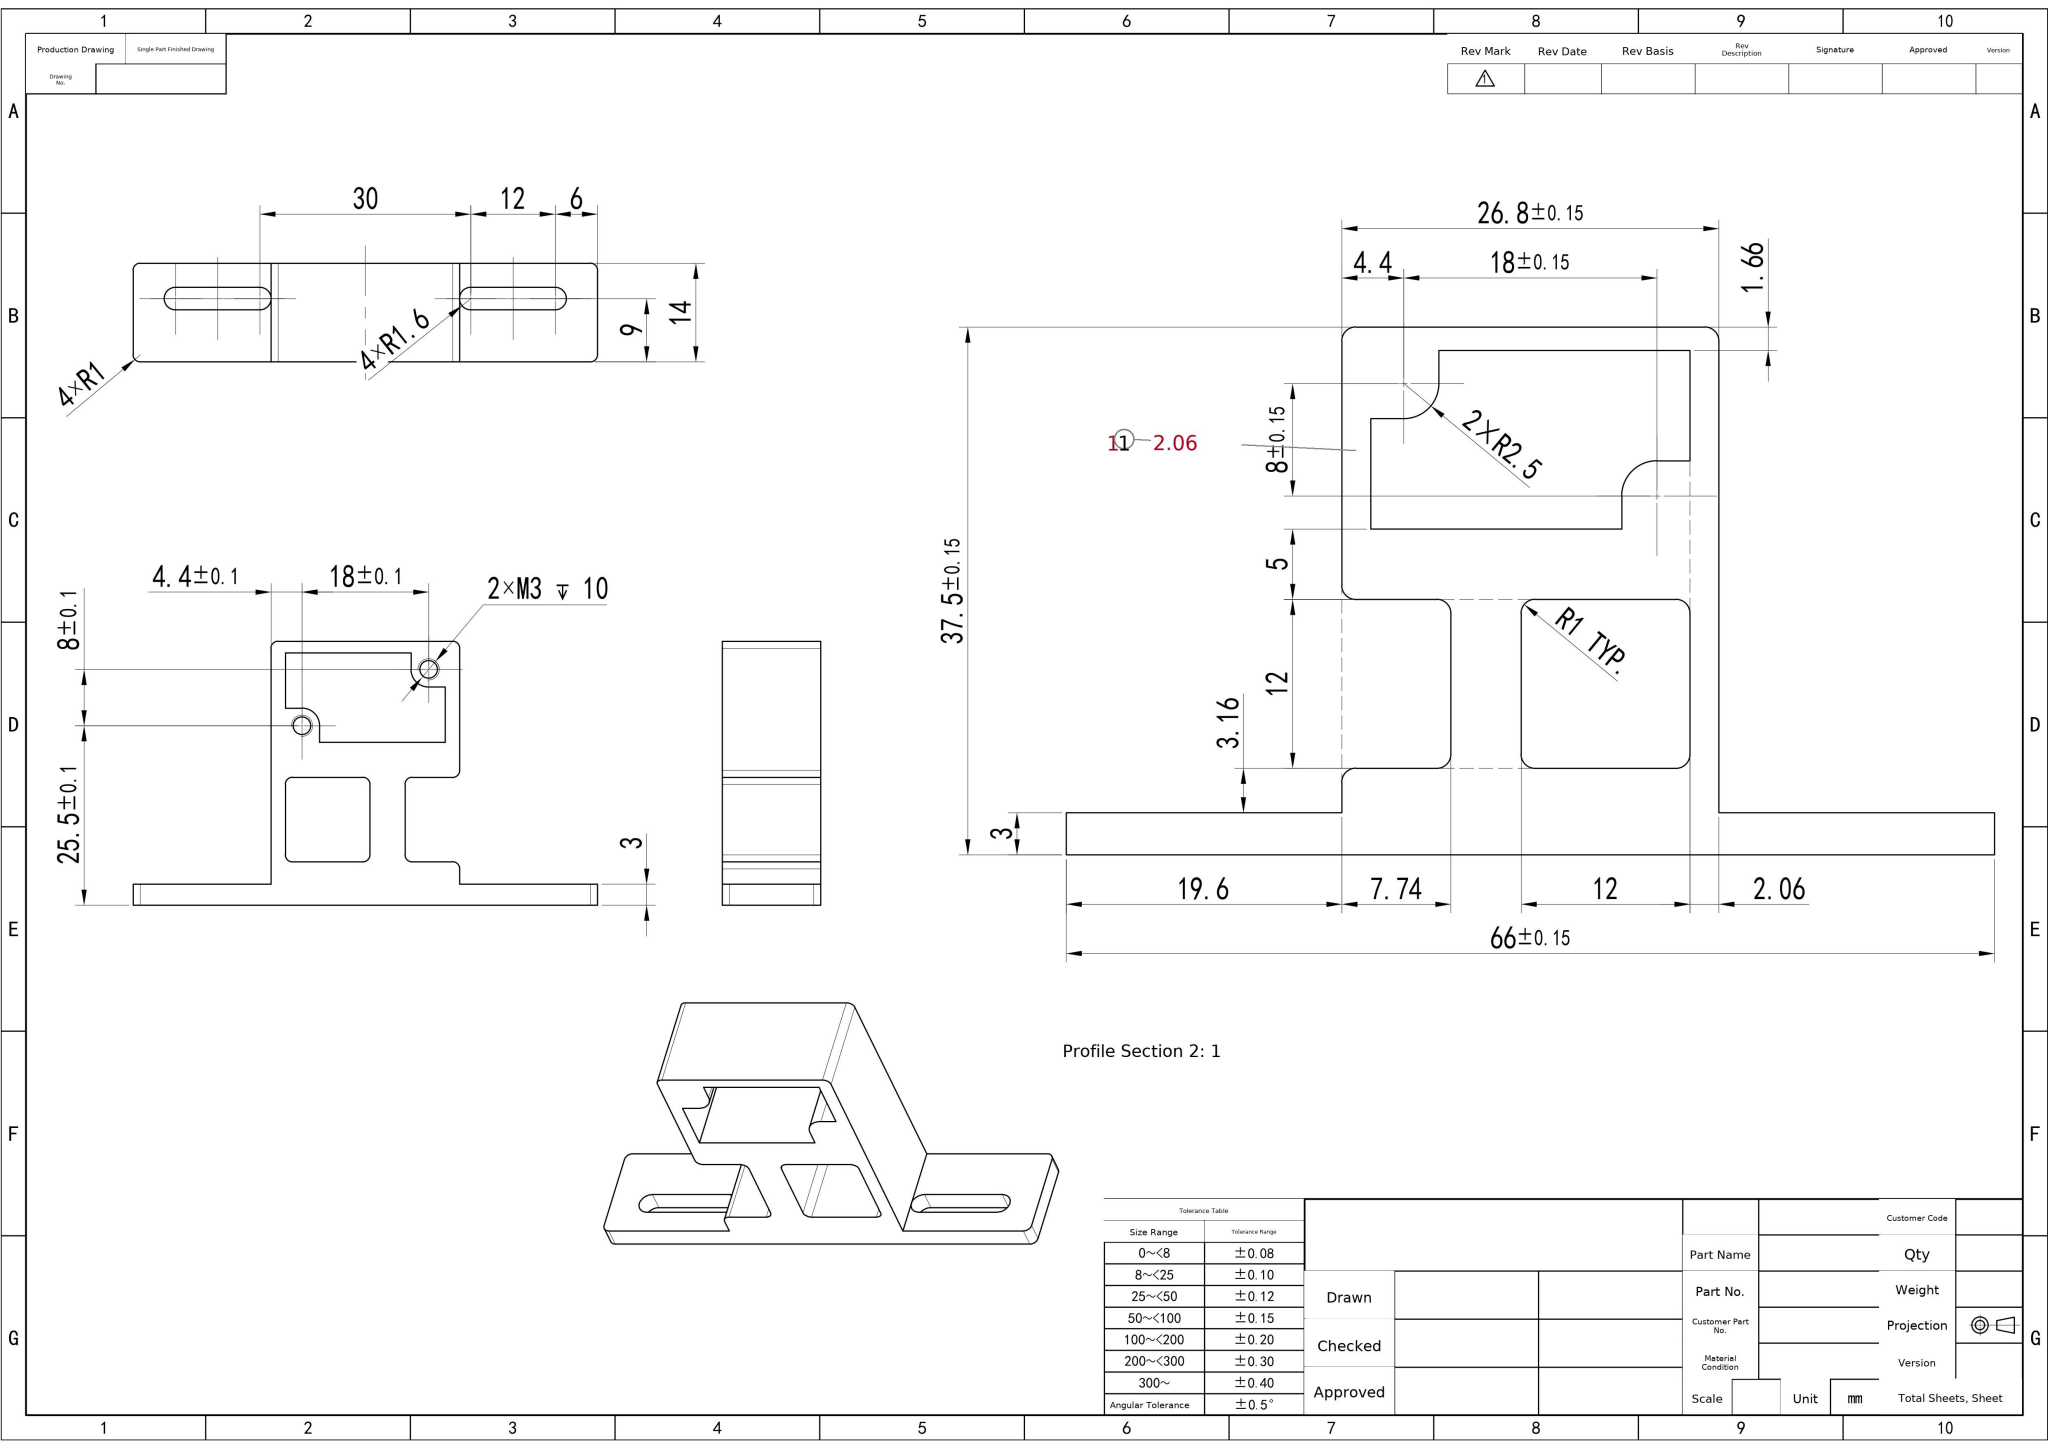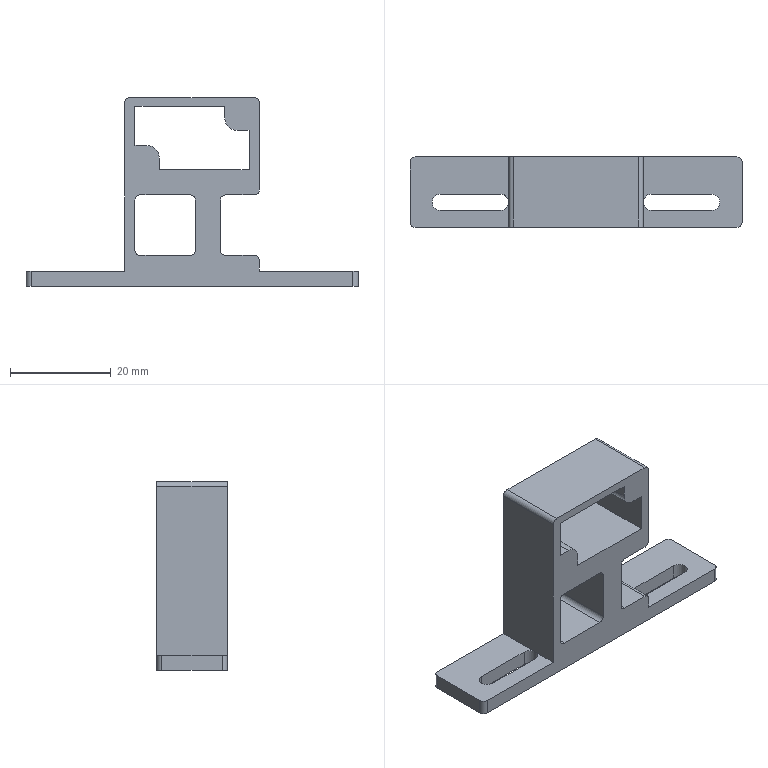Part | SolidWorks | mm | 1 solid | 60 faces | box 66 x 14 x 37.5 mm | volume 8613 mm3 | plane 30 | cylinder 26 | cone 4 | commonest cylinder face diameters 2 x14 3.2 x6 2.5 x4 5 x2